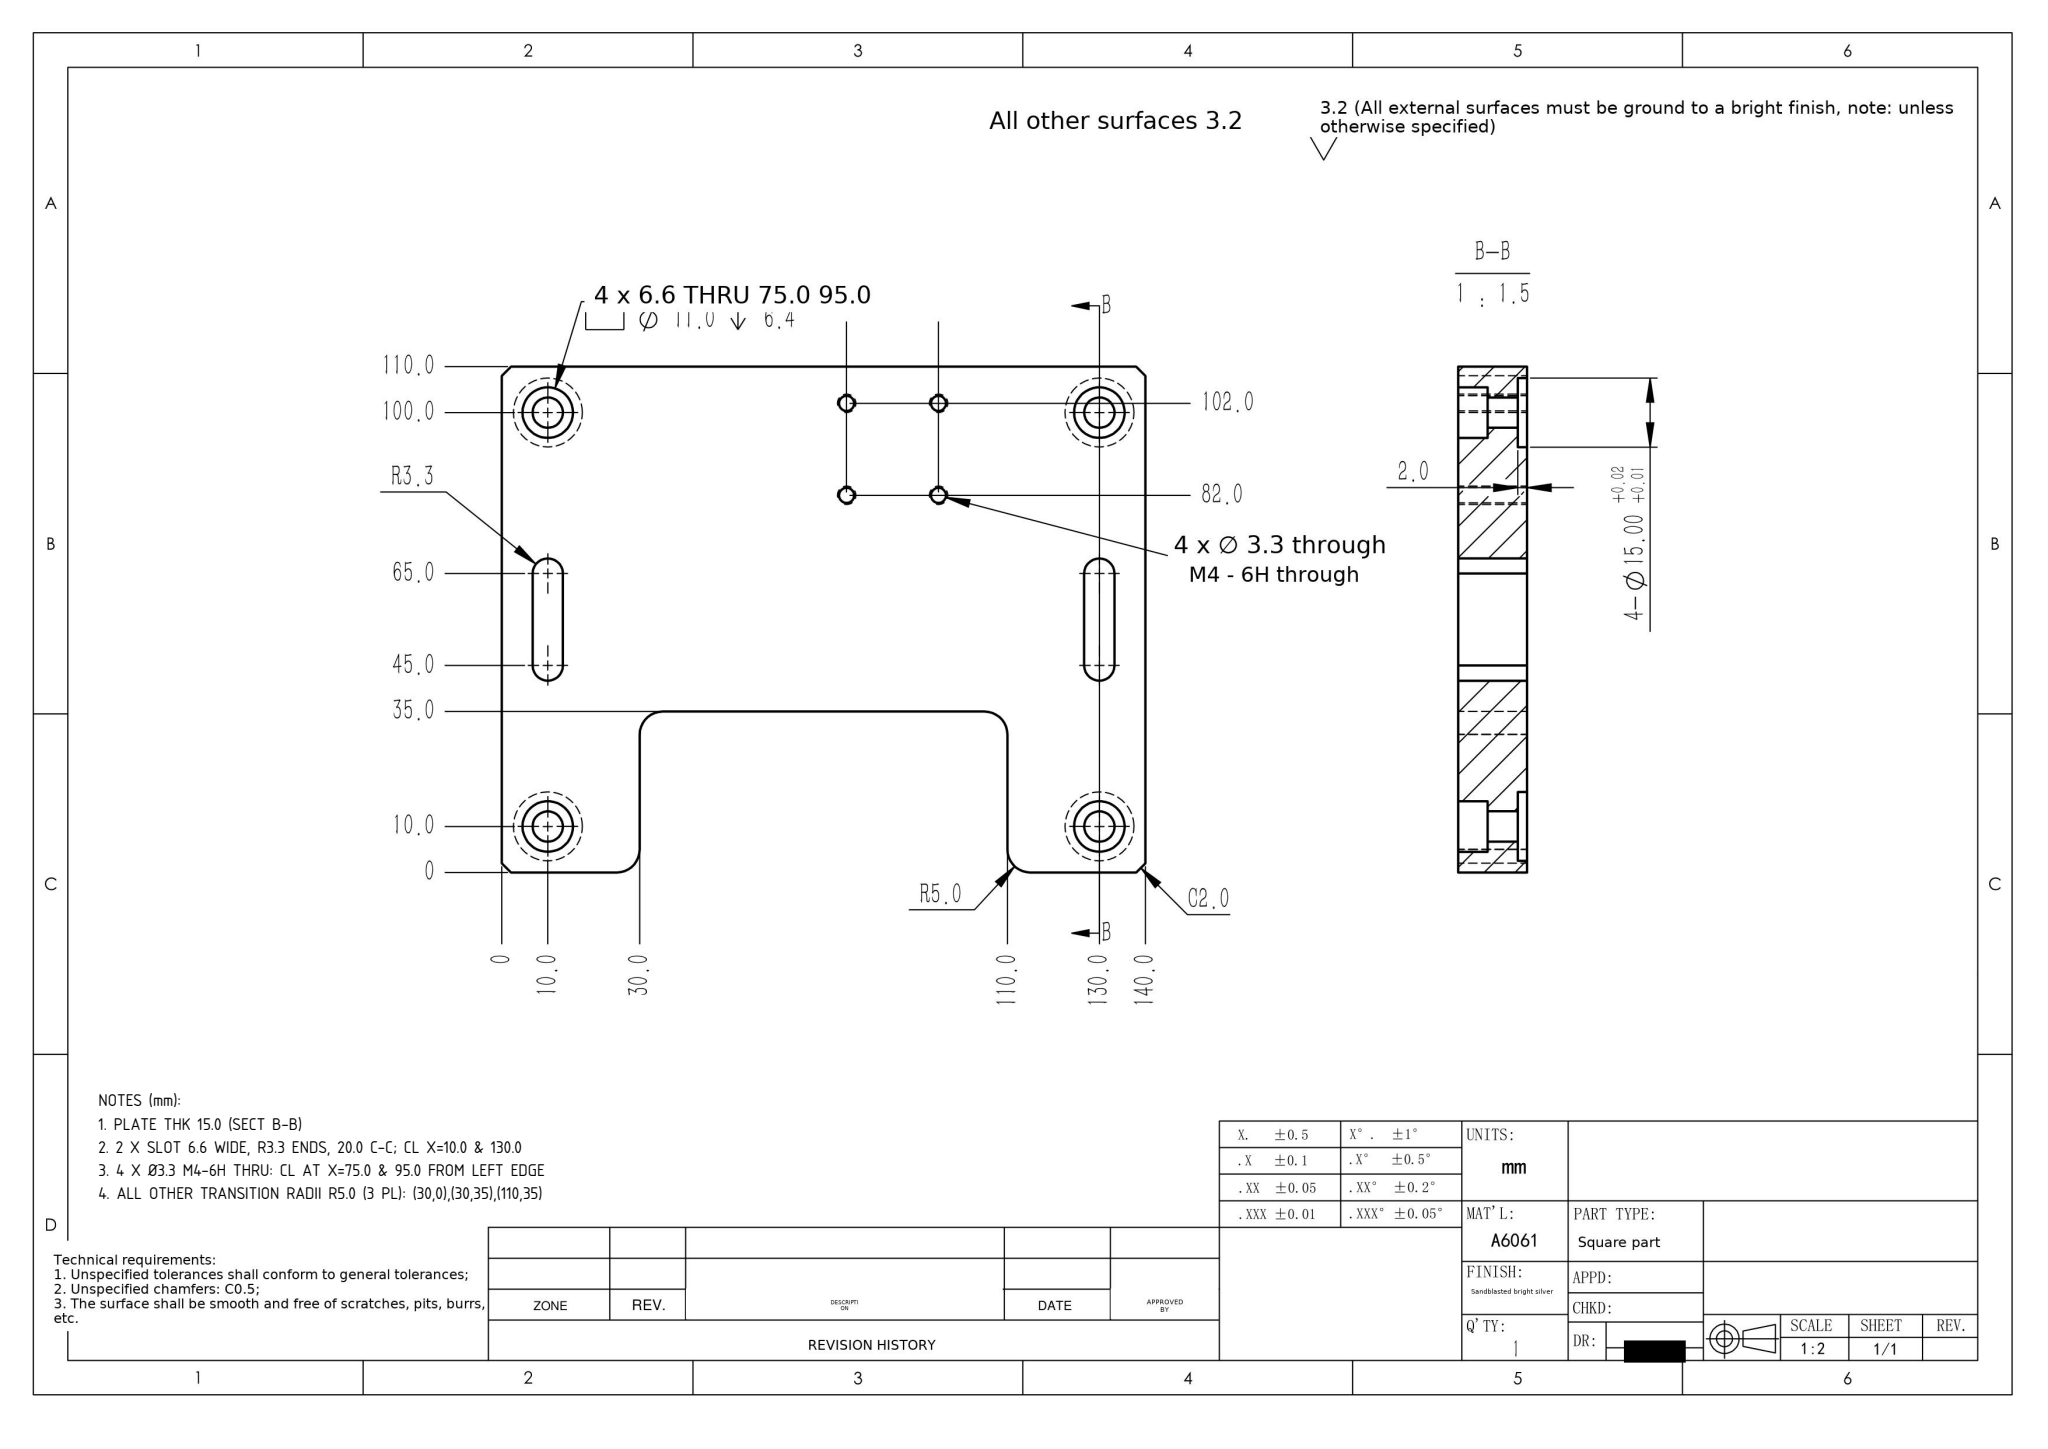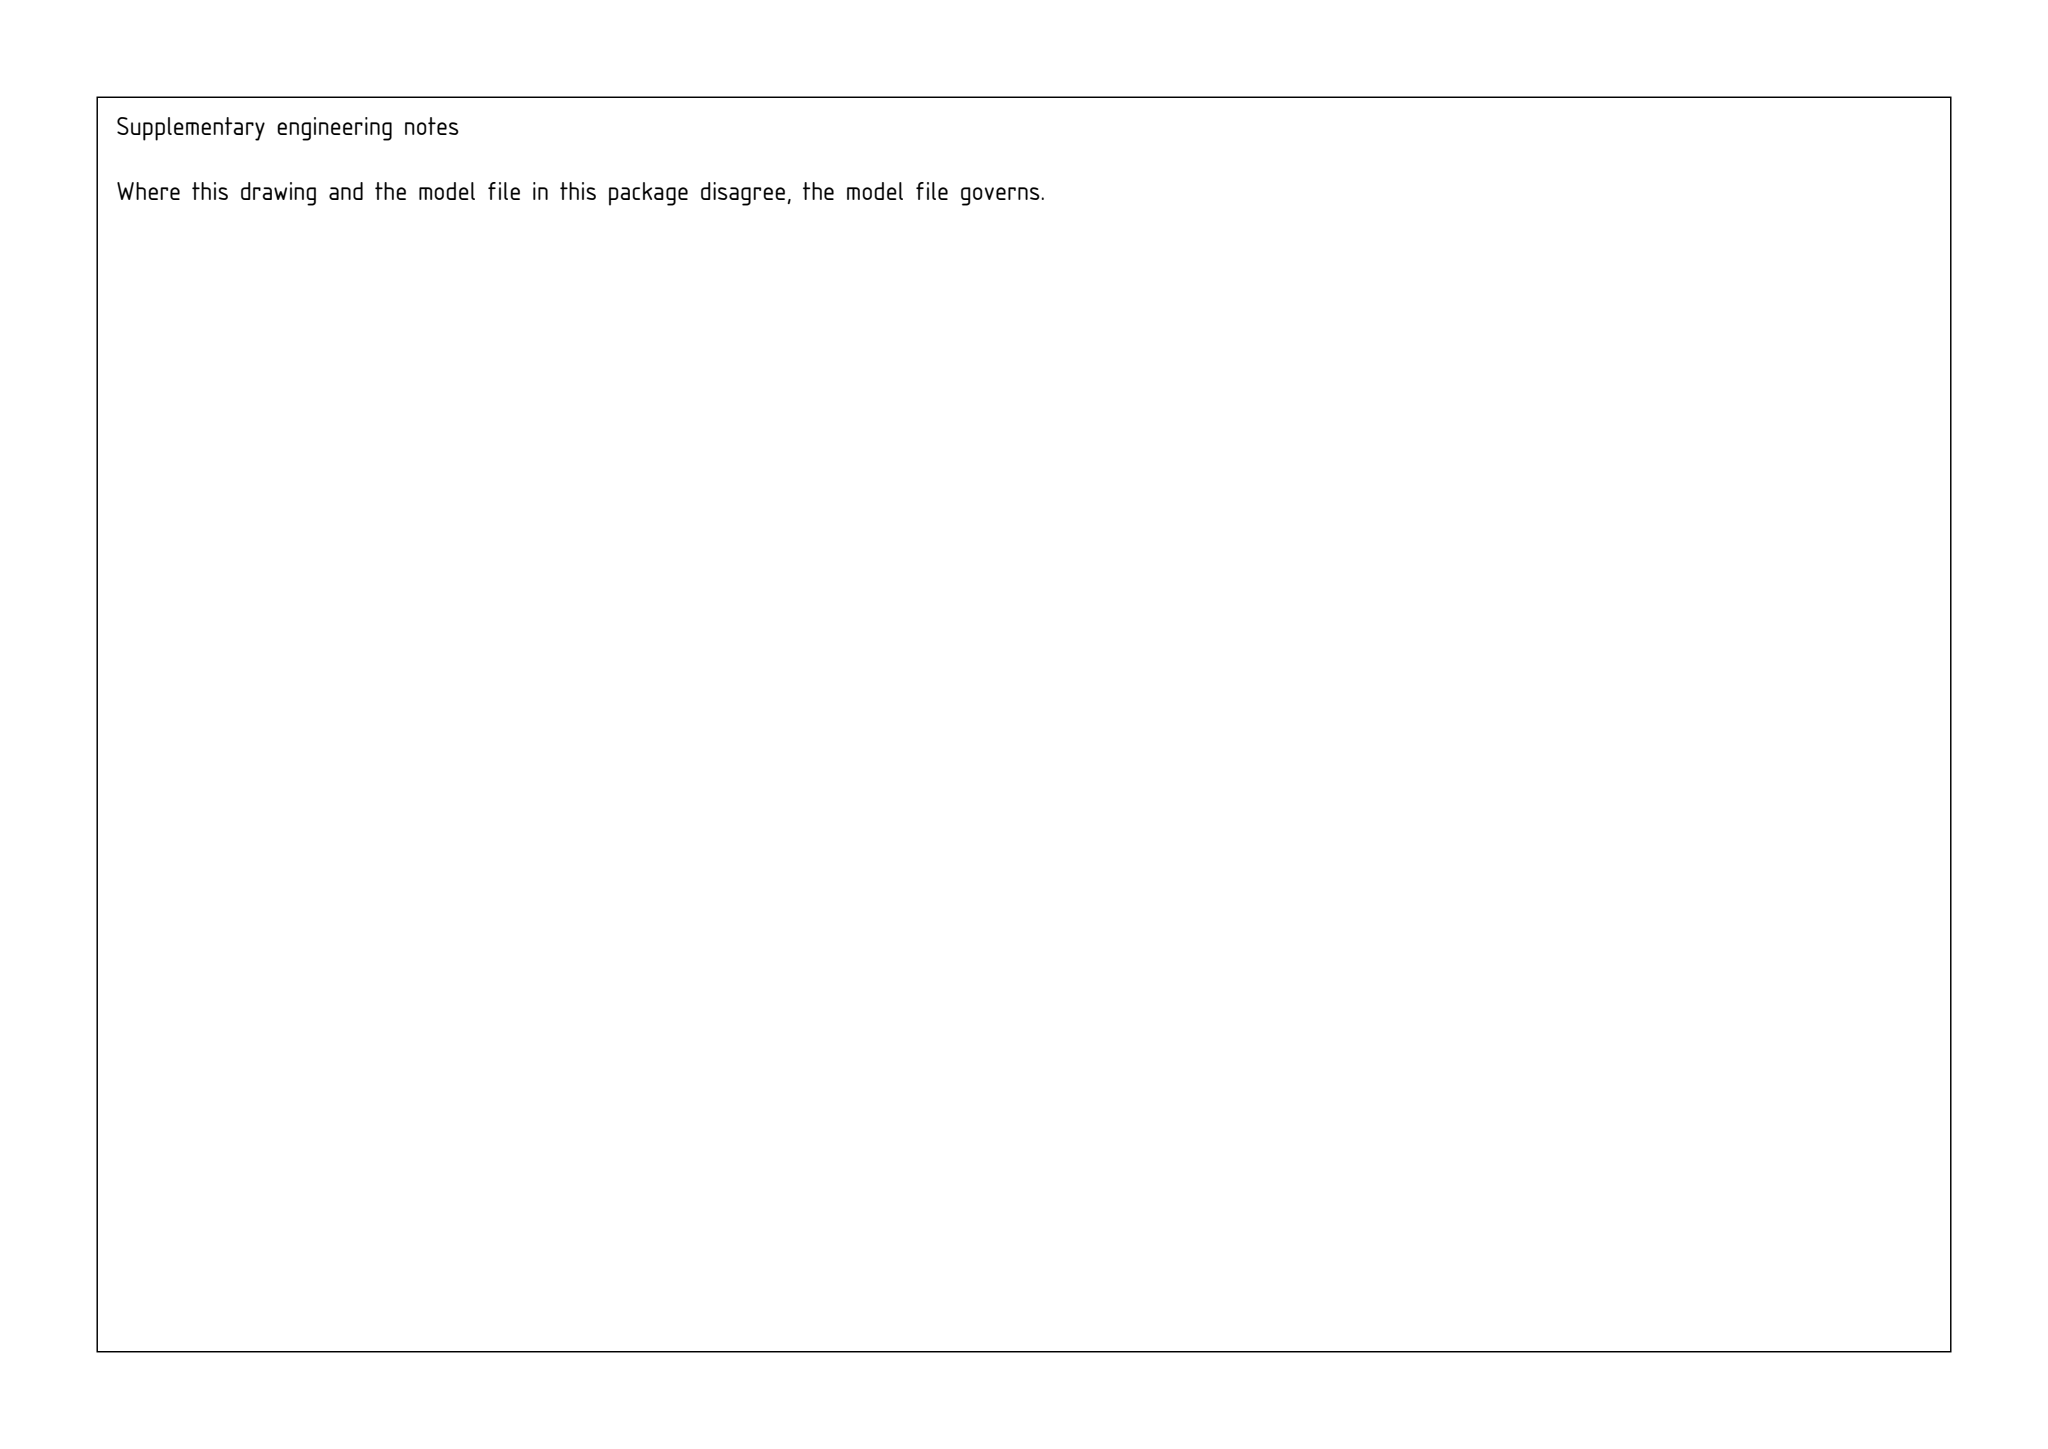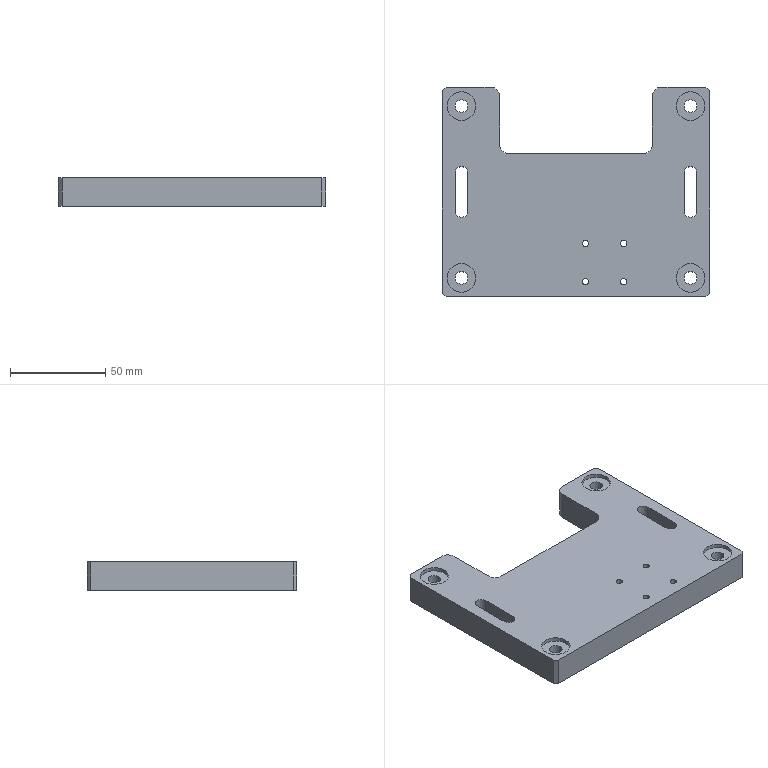Part | SolidWorks | mm | 1 solid | 66 faces | box 140 x 110 x 15 mm | volume 178631 mm3 | cylinder 40 | plane 26 | commonest cylinder face diameters 6.6 x12 3.3 x8 15 x8 11 x8 10 x4
Drawing notes:
PLATE THK 15.0 (SECT B-B) | from the solid: bbox_xyz z = 15.0; z planes at 0.0 and 15.0
2 X SLOT 6.6 WIDE, R3.3 ENDS, 20.0 C-C; CL X=10.0 & 130.0 | from the solid: Ø6.6 thru cyls at (10,45),(10,65),(130,45),(130,65); x planes 6.7/13.3 & 126.7/133.3
4 X Ø3.3 M4-6H THRU: CL AT X=75.0 & 95.0 FROM LEFT EDGE | from the solid: Ø3.3 z-cylinders at x=75.0 & 95.0 (y=8.0/28.0 = 102.0/82.0 from top edge)
ALL OTHER TRANSITION RADII R5.0 (3 PL): (30,0),(30,35),(110,35) | from the solid: Cylindrical transitions tangent to planes x=30, x=110, y=0, y=35 match the called-out R5.0 round at (110,0); 4 total R5 transitions in model
build123d program:
from build123d import *

# Parameters (mm, degrees)
SKETCH1_W                                       = 140
SKETCH1_H                                       = 110
BOSS_EXTRUDE1_DEPTH                             = 15
M6_HEX_SOCKET_HEAD_CAP_SCREW_CBORE1_D           = 6.6
M6_HEX_SOCKET_HEAD_CAP_SCREW_CBORE1_CBORE_D     = 11
M6_HEX_SOCKET_HEAD_CAP_SCREW_CBORE1_CBORE_DEPTH = 6.4
SKETCH4_R                                       = 7.5
CUT_EXTRUDE1_DEPTH                              = 2
SKETCH5_W                                       = 80
SKETCH5_H                                       = 35
CUT_EXTRUDE2_DEPTH                              = 91.277
CUT_EXTRUDE3_DEPTH                              = 91.277
M4_TAPPED_HOLE1_D                               = 3.3
CHAMFER1_SIZE                                   = 2
FILLET1_R                                       = 5


with BuildPart() as part:
    # Sketch1 → Boss-Extrude1 (new body)
    with BuildSketch(Plane.XY):
        Rectangle(SKETCH1_W, SKETCH1_H)
    extrude(amount=BOSS_EXTRUDE1_DEPTH)

    # M6 Hex Socket Head Cap Screw CBORE1 (through all)
    with Locations(Plane(origin=(0, 0, 0), x_dir=(-1, 0, 0), z_dir=(0, 0, -1))):
        with Locations((-60, 45), (60, 45), (60, -45), (-60, -45)):
            CounterBoreHole(M6_HEX_SOCKET_HEAD_CAP_SCREW_CBORE1_D / 2, M6_HEX_SOCKET_HEAD_CAP_SCREW_CBORE1_CBORE_D / 2, M6_HEX_SOCKET_HEAD_CAP_SCREW_CBORE1_CBORE_DEPTH)

    # Sketch4 → Cut-Extrude1 (cut)
    with BuildSketch(Plane.XY.offset(15)):
        with Locations((-60, 45)):
            Circle(SKETCH4_R)
        with Locations((60, 45)):
            Circle(SKETCH4_R)
        with Locations((60, -45)):
            Circle(SKETCH4_R)
        with Locations((-60, -45)):
            Circle(SKETCH4_R)
    extrude(amount=-CUT_EXTRUDE1_DEPTH, mode=Mode.SUBTRACT)

    # Sketch5 → Cut-Extrude2 (cut, through all)
    with BuildSketch(Plane.XY.offset(15)):
        with Locations((0, 37.5)):
            Rectangle(SKETCH5_W, SKETCH5_H)
    extrude(amount=-CUT_EXTRUDE2_DEPTH, mode=Mode.SUBTRACT)

    # Sketch6 → Cut-Extrude3 (cut, through all)
    with BuildSketch(Plane.XY.offset(15)):
        with BuildLine():
            Line((63.3, 10), (63.3, -10))
            ThreePointArc((63.3, -10), (60, -13.3), (56.7, -10))
            Line((56.7, -10), (56.7, 10))
            ThreePointArc((56.7, 10), (60, 13.3), (63.3, 10))
        make_face()
        with BuildLine():
            Line((-56.7, 10), (-56.7, -10))
            ThreePointArc((-56.7, -10), (-60, -13.3), (-63.3, -10))
            Line((-63.3, -10), (-63.3, 10))
            ThreePointArc((-63.3, 10), (-60, 13.3), (-56.7, 10))
        make_face()
    extrude(amount=-CUT_EXTRUDE3_DEPTH, mode=Mode.SUBTRACT)

    # M4 Tapped Hole1 (through all)
    with Locations(Plane.XY.offset(15)):
        with Locations((5, -47), (25, -47), (5, -27), (25, -27)):
            Hole(M4_TAPPED_HOLE1_D / 2)

    # Chamfer1
    chamfer1_edges = [part.edges().sort_by_distance(p)[0] for p in [
        (70, -55, 7.5),
        (-70, -55, 7.5),
        (-70, 55, 7.5),
        (70, 55, 7.5),
    ]]
    chamfer(chamfer1_edges, length=CHAMFER1_SIZE)

    # Fillet1
    fillet1_edges = [part.edges().sort_by_distance(p)[0] for p in [
        (40, 55, 7.5),
        (40, 20, 7.5),
        (-40, 20, 7.5),
        (-40, 55, 7.5),
    ]]
    fillet(fillet1_edges, radius=FILLET1_R)


solid = part.part